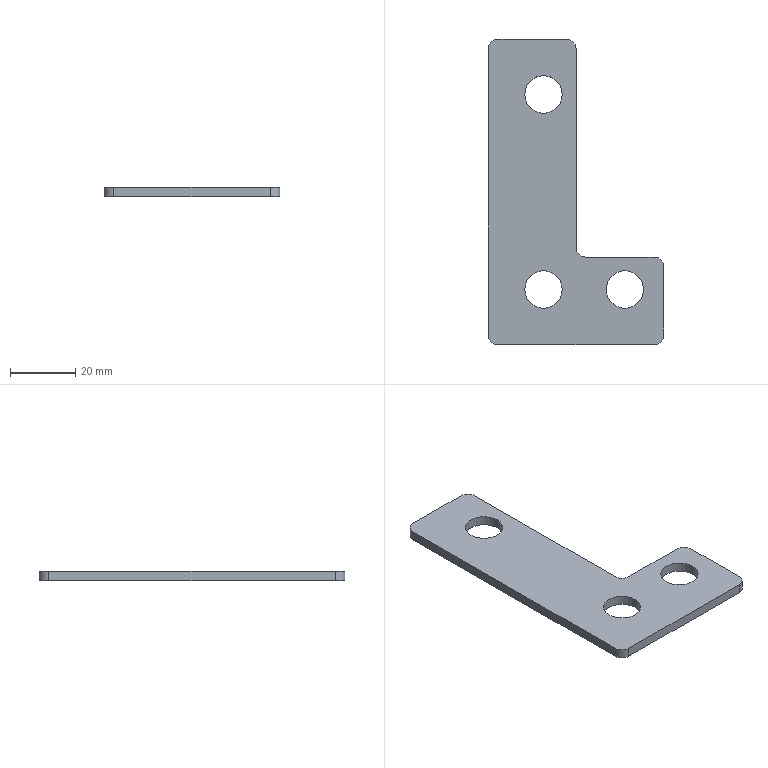Component | SolidWorks | BottomBeamAssembly-1_BottomFrameCornerConnection-1 | 1 solid | 20 faces | box 54 x 94 x 3 mm | volume 8843 mm3 | cylinder 12 | plane 8 | commonest cylinder face diameters 11.5 x6 6 x6
STEP:
#1=COLOUR_RGB('',0.7922,0.8196,0.9333);
#2=FILL_AREA_STYLE_COLOUR('',#1);
#3=FILL_AREA_STYLE('',(#2));
#4=SURFACE_STYLE_FILL_AREA(#3);
#5=SURFACE_SIDE_STYLE('',(#4));
#6=SURFACE_STYLE_USAGE(.BOTH.,#5);
#7=PRESENTATION_STYLE_ASSIGNMENT((#6));
#8=CARTESIAN_POINT('',(-15.865,3.035,-21.339));
#9=VERTEX_POINT('',#8);
#10=CARTESIAN_POINT('',(-15.412,3.035,-21.339));
#11=VERTEX_POINT('',#10);
#12=CARTESIAN_POINT('',(-15.638,3.035,-21.339));
#13=DIRECTION('',(0.,0.,1.));
#14=DIRECTION('',(1.,0.,0.));
#15=AXIS2_PLACEMENT_3D('',#12,#13,#14);
#16=CIRCLE('',#15,0.2264);
#17=EDGE_CURVE('',#9,#11,#16,.T.);
#18=ORIENTED_EDGE('',*,*,#17,.F.);
#19=CARTESIAN_POINT('',(-15.865,3.035,-21.22));
#20=VERTEX_POINT('',#19);
#21=CARTESIAN_POINT('',(-15.865,3.035,-21.614));
#22=DIRECTION('',(0.,0.,1.));
#23=VECTOR('',#22,39.37);
#24=LINE('',#21,#23);
#25=EDGE_CURVE('',#9,#20,#24,.T.);
#26=ORIENTED_EDGE('',*,*,#25,.T.);
#27=CARTESIAN_POINT('',(-15.412,3.035,-21.22));
#28=VERTEX_POINT('',#27);
#29=CARTESIAN_POINT('',(-15.638,3.035,-21.22));
#30=DIRECTION('',(0.,0.,1.));
#31=DIRECTION('',(1.,0.,0.));
#32=AXIS2_PLACEMENT_3D('',#29,#30,#31);
#33=CIRCLE('',#32,0.2264);
#34=EDGE_CURVE('',#20,#28,#33,.T.);
#35=ORIENTED_EDGE('',*,*,#34,.T.);
#36=CARTESIAN_POINT('',(-15.412,3.035,-21.614));
#37=DIRECTION('',(0.,0.,1.));
#38=VECTOR('',#37,39.37);
#39=LINE('',#36,#38);
#40=EDGE_CURVE('',#11,#28,#39,.T.);
#41=ORIENTED_EDGE('',*,*,#40,.F.);
#42=EDGE_LOOP('',(#18,#26,#35,#41));
#43=FACE_OUTER_BOUND('',#42,.T.);
#44=CARTESIAN_POINT('',(-15.638,3.035,-21.614));
#45=DIRECTION('',(0.,0.,1.));
#46=DIRECTION('',(1.,0.,0.));
#47=AXIS2_PLACEMENT_3D('',#44,#45,#46);
#48=CYLINDRICAL_SURFACE('',#47,0.2264);
#49=ADVANCED_FACE('',(#43),#48,.F.);
#50=CARTESIAN_POINT('',(-14.881,0.6732,-21.339));
#51=VERTEX_POINT('',#50);
#52=CARTESIAN_POINT('',(-14.428,0.6732,-21.339));
#53=VERTEX_POINT('',#52);
#54=CARTESIAN_POINT('',(-14.654,0.6732,-21.339));
#55=DIRECTION('',(0.,0.,1.));
#56=DIRECTION('',(1.,0.,0.));
#57=AXIS2_PLACEMENT_3D('',#54,#55,#56);
#58=CIRCLE('',#57,0.2264);
#59=EDGE_CURVE('',#51,#53,#58,.T.);
#60=ORIENTED_EDGE('',*,*,#59,.F.);
#61=CARTESIAN_POINT('',(-14.881,0.6732,-21.22));
#62=VERTEX_POINT('',#61);
#63=CARTESIAN_POINT('',(-14.881,0.6732,-21.614));
#64=DIRECTION('',(0.,0.,1.));
#65=VECTOR('',#64,39.37);
#66=LINE('',#63,#65);
#67=EDGE_CURVE('',#51,#62,#66,.T.);
#68=ORIENTED_EDGE('',*,*,#67,.T.);
#69=CARTESIAN_POINT('',(-14.428,0.6732,-21.22));
#70=VERTEX_POINT('',#69);
#71=CARTESIAN_POINT('',(-14.654,0.6732,-21.22));
#72=DIRECTION('',(0.,0.,1.));
#73=DIRECTION('',(1.,0.,0.));
#74=AXIS2_PLACEMENT_3D('',#71,#72,#73);
#75=CIRCLE('',#74,0.2264);
#76=EDGE_CURVE('',#62,#70,#75,.T.);
#77=ORIENTED_EDGE('',*,*,#76,.T.);
#78=CARTESIAN_POINT('',(-14.428,0.6732,-21.614));
#79=DIRECTION('',(0.,0.,1.));
#80=VECTOR('',#79,39.37);
#81=LINE('',#78,#80);
#82=EDGE_CURVE('',#53,#70,#81,.T.);
#83=ORIENTED_EDGE('',*,*,#82,.F.);
#84=EDGE_LOOP('',(#60,#68,#77,#83));
#85=FACE_OUTER_BOUND('',#84,.T.);
#86=CARTESIAN_POINT('',(-14.654,0.6732,-21.614));
#87=DIRECTION('',(0.,0.,1.));
#88=DIRECTION('',(1.,0.,0.));
#89=AXIS2_PLACEMENT_3D('',#86,#87,#88);
#90=CYLINDRICAL_SURFACE('',#89,0.2264);
#91=ADVANCED_FACE('',(#85),#90,.F.);
#92=CARTESIAN_POINT('',(-15.865,0.6732,-21.339));
#93=VERTEX_POINT('',#92);
#94=CARTESIAN_POINT('',(-15.412,0.6732,-21.339));
#95=VERTEX_POINT('',#94);
#96=CARTESIAN_POINT('',(-15.638,0.6732,-21.339));
#97=DIRECTION('',(0.,0.,1.));
#98=DIRECTION('',(1.,0.,0.));
#99=AXIS2_PLACEMENT_3D('',#96,#97,#98);
#100=CIRCLE('',#99,0.2264);
#101=EDGE_CURVE('',#93,#95,#100,.T.);
#102=ORIENTED_EDGE('',*,*,#101,.F.);
#103=CARTESIAN_POINT('',(-15.865,0.6732,-21.22));
#104=VERTEX_POINT('',#103);
#105=CARTESIAN_POINT('',(-15.865,0.6732,-21.614));
#106=DIRECTION('',(0.,0.,1.));
#107=VECTOR('',#106,39.37);
#108=LINE('',#105,#107);
#109=EDGE_CURVE('',#93,#104,#108,.T.);
#110=ORIENTED_EDGE('',*,*,#109,.T.);
#111=CARTESIAN_POINT('',(-15.412,0.6732,-21.22));
#112=VERTEX_POINT('',#111);
#113=CARTESIAN_POINT('',(-15.638,0.6732,-21.22));
#114=DIRECTION('',(0.,0.,1.));
#115=DIRECTION('',(1.,0.,0.));
#116=AXIS2_PLACEMENT_3D('',#113,#114,#115);
#117=CIRCLE('',#116,0.2264);
#118=EDGE_CURVE('',#104,#112,#117,.T.);
#119=ORIENTED_EDGE('',*,*,#118,.T.);
#120=CARTESIAN_POINT('',(-15.412,0.6732,-21.614));
#121=DIRECTION('',(0.,0.,1.));
#122=VECTOR('',#121,39.37);
#123=LINE('',#120,#122);
#124=EDGE_CURVE('',#95,#112,#123,.T.);
#125=ORIENTED_EDGE('',*,*,#124,.F.);
#126=EDGE_LOOP('',(#102,#110,#119,#125));
#127=FACE_OUTER_BOUND('',#126,.T.);
#128=CARTESIAN_POINT('',(-15.638,0.6732,-21.614));
#129=DIRECTION('',(0.,0.,1.));
#130=DIRECTION('',(1.,0.,0.));
#131=AXIS2_PLACEMENT_3D('',#128,#129,#130);
#132=CYLINDRICAL_SURFACE('',#131,0.2264);
#133=ADVANCED_FACE('',(#127),#132,.F.);
#134=CARTESIAN_POINT('',(-16.308,3.587,-21.339));
#135=VERTEX_POINT('',#134);
#136=CARTESIAN_POINT('',(-16.308,0.122,-21.339));
#137=VERTEX_POINT('',#136);
#138=CARTESIAN_POINT('',(-16.308,3.705,-21.339));
#139=DIRECTION('',(0.,-1.,0.));
#140=VECTOR('',#139,39.37);
#141=LINE('',#138,#140);
#142=EDGE_CURVE('',#135,#137,#141,.T.);
#143=ORIENTED_EDGE('',*,*,#142,.T.);
#144=CARTESIAN_POINT('',(-16.308,0.122,-21.22));
#145=VERTEX_POINT('',#144);
#146=CARTESIAN_POINT('',(-16.308,0.122,-21.339));
#147=DIRECTION('',(0.,0.,1.));
#148=VECTOR('',#147,39.37);
#149=LINE('',#146,#148);
#150=EDGE_CURVE('',#137,#145,#149,.T.);
#151=ORIENTED_EDGE('',*,*,#150,.T.);
#152=CARTESIAN_POINT('',(-16.308,3.587,-21.22));
#153=VERTEX_POINT('',#152);
#154=CARTESIAN_POINT('',(-16.308,3.705,-21.22));
#155=DIRECTION('',(0.,-1.,0.));
#156=VECTOR('',#155,39.37);
#157=LINE('',#154,#156);
#158=EDGE_CURVE('',#153,#145,#157,.T.);
#159=ORIENTED_EDGE('',*,*,#158,.F.);
#160=CARTESIAN_POINT('',(-16.308,3.587,-21.339));
#161=DIRECTION('',(0.,0.,-1.));
#162=VECTOR('',#161,39.37);
#163=LINE('',#160,#162);
#164=EDGE_CURVE('',#153,#135,#163,.T.);
#165=ORIENTED_EDGE('',*,*,#164,.T.);
#166=EDGE_LOOP('',(#143,#151,#159,#165));
#167=FACE_OUTER_BOUND('',#166,.T.);
#168=CARTESIAN_POINT('',(-16.308,3.705,-21.339));
#169=DIRECTION('',(-1.,-0.,0.));
#170=DIRECTION('',(0.,-1.,0.));
#171=AXIS2_PLACEMENT_3D('',#168,#169,#170);
#172=PLANE('',#171);
#173=ADVANCED_FACE('',(#167),#172,.T.);
#174=CARTESIAN_POINT('',(-15.363,3.705,-21.22));
#175=VERTEX_POINT('',#174);
#176=CARTESIAN_POINT('',(-16.19,3.705,-21.22));
#177=VERTEX_POINT('',#176);
#178=CARTESIAN_POINT('',(-15.245,3.705,-21.22));
#179=DIRECTION('',(-1.,0.,0.));
#180=VECTOR('',#179,39.37);
#181=LINE('',#178,#180);
#182=EDGE_CURVE('',#175,#177,#181,.T.);
#183=ORIENTED_EDGE('',*,*,#182,.F.);
#184=CARTESIAN_POINT('',(-15.363,3.705,-21.339));
#185=VERTEX_POINT('',#184);
#186=CARTESIAN_POINT('',(-15.363,3.705,-21.339));
#187=DIRECTION('',(0.,0.,-1.));
#188=VECTOR('',#187,39.37);
#189=LINE('',#186,#188);
#190=EDGE_CURVE('',#175,#185,#189,.T.);
#191=ORIENTED_EDGE('',*,*,#190,.T.);
#192=CARTESIAN_POINT('',(-16.19,3.705,-21.339));
#193=VERTEX_POINT('',#192);
#194=CARTESIAN_POINT('',(-15.245,3.705,-21.339));
#195=DIRECTION('',(-1.,0.,0.));
#196=VECTOR('',#195,39.37);
#197=LINE('',#194,#196);
#198=EDGE_CURVE('',#185,#193,#197,.T.);
#199=ORIENTED_EDGE('',*,*,#198,.T.);
#200=CARTESIAN_POINT('',(-16.19,3.705,-21.339));
#201=DIRECTION('',(0.,0.,1.));
#202=VECTOR('',#201,39.37);
#203=LINE('',#200,#202);
#204=EDGE_CURVE('',#193,#177,#203,.T.);
#205=ORIENTED_EDGE('',*,*,#204,.T.);
#206=EDGE_LOOP('',(#183,#191,#199,#205));
#207=FACE_OUTER_BOUND('',#206,.T.);
#208=CARTESIAN_POINT('',(-15.245,3.705,-21.339));
#209=DIRECTION('',(0.,1.,0.));
#210=DIRECTION('',(0.,0.,1.));
#211=AXIS2_PLACEMENT_3D('',#208,#209,#210);
#212=PLANE('',#211);
#213=ADVANCED_FACE('',(#207),#212,.T.);
#214=CARTESIAN_POINT('',(-15.245,1.185,-21.22));
#215=VERTEX_POINT('',#214);
#216=CARTESIAN_POINT('',(-15.245,3.587,-21.22));
#217=VERTEX_POINT('',#216);
#218=CARTESIAN_POINT('',(-15.245,1.067,-21.22));
#219=DIRECTION('',(0.,1.,0.));
#220=VECTOR('',#219,39.37);
#221=LINE('',#218,#220);
#222=EDGE_CURVE('',#215,#217,#221,.T.);
#223=ORIENTED_EDGE('',*,*,#222,.F.);
#224=CARTESIAN_POINT('',(-15.245,1.185,-21.339));
#225=VERTEX_POINT('',#224);
#226=CARTESIAN_POINT('',(-15.245,1.185,-21.339));
#227=DIRECTION('',(0.,0.,-1.));
#228=VECTOR('',#227,39.37);
#229=LINE('',#226,#228);
#230=EDGE_CURVE('',#215,#225,#229,.T.);
#231=ORIENTED_EDGE('',*,*,#230,.T.);
#232=CARTESIAN_POINT('',(-15.245,3.587,-21.339));
#233=VERTEX_POINT('',#232);
#234=CARTESIAN_POINT('',(-15.245,1.067,-21.339));
#235=DIRECTION('',(0.,1.,0.));
#236=VECTOR('',#235,39.37);
#237=LINE('',#234,#236);
#238=EDGE_CURVE('',#225,#233,#237,.T.);
#239=ORIENTED_EDGE('',*,*,#238,.T.);
#240=CARTESIAN_POINT('',(-15.245,3.587,-21.339));
#241=DIRECTION('',(0.,0.,1.));
#242=VECTOR('',#241,39.37);
#243=LINE('',#240,#242);
#244=EDGE_CURVE('',#233,#217,#243,.T.);
#245=ORIENTED_EDGE('',*,*,#244,.T.);
#246=EDGE_LOOP('',(#223,#231,#239,#245));
#247=FACE_OUTER_BOUND('',#246,.T.);
#248=CARTESIAN_POINT('',(-15.245,1.067,-21.339));
#249=DIRECTION('',(1.,0.,0.));
#250=DIRECTION('',(0.,0.,-1.));
#251=AXIS2_PLACEMENT_3D('',#248,#249,#250);
#252=PLANE('',#251);
#253=ADVANCED_FACE('',(#247),#252,.T.);
#254=CARTESIAN_POINT('',(-14.3,1.067,-21.339));
#255=VERTEX_POINT('',#254);
#256=CARTESIAN_POINT('',(-15.127,1.067,-21.339));
#257=VERTEX_POINT('',#256);
#258=CARTESIAN_POINT('',(-14.182,1.067,-21.339));
#259=DIRECTION('',(-1.,-0.,0.));
#260=VECTOR('',#259,39.37);
#261=LINE('',#258,#260);
#262=EDGE_CURVE('',#255,#257,#261,.T.);
#263=ORIENTED_EDGE('',*,*,#262,.T.);
#264=CARTESIAN_POINT('',(-15.127,1.067,-21.22));
#265=VERTEX_POINT('',#264);
#266=CARTESIAN_POINT('',(-15.127,1.067,-21.22));
#267=DIRECTION('',(0.,0.,1.));
#268=VECTOR('',#267,39.37);
#269=LINE('',#266,#268);
#270=EDGE_CURVE('',#257,#265,#269,.T.);
#271=ORIENTED_EDGE('',*,*,#270,.T.);
#272=CARTESIAN_POINT('',(-14.3,1.067,-21.22));
#273=VERTEX_POINT('',#272);
#274=CARTESIAN_POINT('',(-14.182,1.067,-21.22));
#275=DIRECTION('',(-1.,-0.,0.));
#276=VECTOR('',#275,39.37);
#277=LINE('',#274,#276);
#278=EDGE_CURVE('',#273,#265,#277,.T.);
#279=ORIENTED_EDGE('',*,*,#278,.F.);
#280=CARTESIAN_POINT('',(-14.3,1.067,-21.339));
#281=DIRECTION('',(0.,0.,-1.));
#282=VECTOR('',#281,39.37);
#283=LINE('',#280,#282);
#284=EDGE_CURVE('',#273,#255,#283,.T.);
#285=ORIENTED_EDGE('',*,*,#284,.T.);
#286=EDGE_LOOP('',(#263,#271,#279,#285));
#287=FACE_OUTER_BOUND('',#286,.T.);
#288=CARTESIAN_POINT('',(-14.182,1.067,-21.339));
#289=DIRECTION('',(-0.,1.,0.));
#290=DIRECTION('',(-1.,-0.,0.));
#291=AXIS2_PLACEMENT_3D('',#288,#289,#290);
#292=PLANE('',#291);
#293=ADVANCED_FACE('',(#287),#292,.T.);
#294=CARTESIAN_POINT('',(-14.182,0.122,-21.22));
#295=VERTEX_POINT('',#294);
#296=CARTESIAN_POINT('',(-14.182,0.9488,-21.22));
#297=VERTEX_POINT('',#296);
#298=CARTESIAN_POINT('',(-14.182,0.003927,-21.22));
#299=DIRECTION('',(0.,1.,0.));
#300=VECTOR('',#299,39.37);
#301=LINE('',#298,#300);
#302=EDGE_CURVE('',#295,#297,#301,.T.);
#303=ORIENTED_EDGE('',*,*,#302,.F.);
#304=CARTESIAN_POINT('',(-14.182,0.122,-21.339));
#305=VERTEX_POINT('',#304);
#306=CARTESIAN_POINT('',(-14.182,0.122,-21.339));
#307=DIRECTION('',(0.,0.,-1.));
#308=VECTOR('',#307,39.37);
#309=LINE('',#306,#308);
#310=EDGE_CURVE('',#295,#305,#309,.T.);
#311=ORIENTED_EDGE('',*,*,#310,.T.);
#312=CARTESIAN_POINT('',(-14.182,0.9488,-21.339));
#313=VERTEX_POINT('',#312);
#314=CARTESIAN_POINT('',(-14.182,0.003927,-21.339));
#315=DIRECTION('',(0.,1.,0.));
#316=VECTOR('',#315,39.37);
#317=LINE('',#314,#316);
#318=EDGE_CURVE('',#305,#313,#317,.T.);
#319=ORIENTED_EDGE('',*,*,#318,.T.);
#320=CARTESIAN_POINT('',(-14.182,0.9488,-21.339));
#321=DIRECTION('',(0.,0.,1.));
#322=VECTOR('',#321,39.37);
#323=LINE('',#320,#322);
#324=EDGE_CURVE('',#313,#297,#323,.T.);
#325=ORIENTED_EDGE('',*,*,#324,.T.);
#326=EDGE_LOOP('',(#303,#311,#319,#325));
#327=FACE_OUTER_BOUND('',#326,.T.);
#328=CARTESIAN_POINT('',(-14.182,0.003927,-21.339));
#329=DIRECTION('',(1.,0.,0.));
#330=DIRECTION('',(0.,0.,-1.));
#331=AXIS2_PLACEMENT_3D('',#328,#329,#330);
#332=PLANE('',#331);
#333=ADVANCED_FACE('',(#327),#332,.T.);
#334=CARTESIAN_POINT('',(-16.19,0.003927,-21.22));
#335=VERTEX_POINT('',#334);
#336=CARTESIAN_POINT('',(-14.3,0.003927,-21.22));
#337=VERTEX_POINT('',#336);
#338=CARTESIAN_POINT('',(-16.308,0.003927,-21.22));
#339=DIRECTION('',(1.,0.,0.));
#340=VECTOR('',#339,39.37);
#341=LINE('',#338,#340);
#342=EDGE_CURVE('',#335,#337,#341,.T.);
#343=ORIENTED_EDGE('',*,*,#342,.F.);
#344=CARTESIAN_POINT('',(-16.19,0.003927,-21.339));
#345=VERTEX_POINT('',#344);
#346=CARTESIAN_POINT('',(-16.19,0.003927,-21.339));
#347=DIRECTION('',(0.,0.,-1.));
#348=VECTOR('',#347,39.37);
#349=LINE('',#346,#348);
#350=EDGE_CURVE('',#335,#345,#349,.T.);
#351=ORIENTED_EDGE('',*,*,#350,.T.);
#352=CARTESIAN_POINT('',(-14.3,0.003927,-21.339));
#353=VERTEX_POINT('',#352);
#354=CARTESIAN_POINT('',(-16.308,0.003927,-21.339));
#355=DIRECTION('',(1.,0.,0.));
#356=VECTOR('',#355,39.37);
#357=LINE('',#354,#356);
#358=EDGE_CURVE('',#345,#353,#357,.T.);
#359=ORIENTED_EDGE('',*,*,#358,.T.);
#360=CARTESIAN_POINT('',(-14.3,0.003927,-21.339));
#361=DIRECTION('',(0.,0.,1.));
#362=VECTOR('',#361,39.37);
#363=LINE('',#360,#362);
#364=EDGE_CURVE('',#353,#337,#363,.T.);
#365=ORIENTED_EDGE('',*,*,#364,.T.);
#366=EDGE_LOOP('',(#343,#351,#359,#365));
#367=FACE_OUTER_BOUND('',#366,.T.);
#368=CARTESIAN_POINT('',(-16.308,0.003927,-21.339));
#369=DIRECTION('',(0.,-1.,0.));
#370=DIRECTION('',(0.,0.,-1.));
#371=AXIS2_PLACEMENT_3D('',#368,#369,#370);
#372=PLANE('',#371);
#373=ADVANCED_FACE('',(#367),#372,.T.);
#374=CARTESIAN_POINT('',(-15.638,3.035,-21.339));
#375=DIRECTION('',(0.,0.,1.));
#376=DIRECTION('',(1.,0.,0.));
#377=AXIS2_PLACEMENT_3D('',#374,#375,#376);
#378=CIRCLE('',#377,0.2264);
#379=EDGE_CURVE('',#11,#9,#378,.T.);
#380=ORIENTED_EDGE('',*,*,#379,.T.);
#381=ORIENTED_EDGE('',*,*,#17,.T.);
#382=EDGE_LOOP('',(#380,#381));
#383=FACE_BOUND('',#382,.T.);
#384=CARTESIAN_POINT('',(-14.654,0.6732,-21.339));
#385=DIRECTION('',(0.,0.,1.));
#386=DIRECTION('',(1.,0.,0.));
#387=AXIS2_PLACEMENT_3D('',#384,#385,#386);
#388=CIRCLE('',#387,0.2264);
#389=EDGE_CURVE('',#53,#51,#388,.T.);
#390=ORIENTED_EDGE('',*,*,#389,.T.);
#391=ORIENTED_EDGE('',*,*,#59,.T.);
#392=EDGE_LOOP('',(#390,#391));
#393=FACE_BOUND('',#392,.T.);
#394=CARTESIAN_POINT('',(-15.638,0.6732,-21.339));
#395=DIRECTION('',(0.,0.,1.));
#396=DIRECTION('',(1.,0.,0.));
#397=AXIS2_PLACEMENT_3D('',#394,#395,#396);
#398=CIRCLE('',#397,0.2264);
#399=EDGE_CURVE('',#95,#93,#398,.T.);
#400=ORIENTED_EDGE('',*,*,#399,.T.);
#401=ORIENTED_EDGE('',*,*,#101,.T.);
#402=EDGE_LOOP('',(#400,#401));
#403=FACE_BOUND('',#402,.T.);
#404=ORIENTED_EDGE('',*,*,#358,.F.);
#405=CARTESIAN_POINT('',(-16.19,0.122,-21.339));
#406=DIRECTION('',(0.,0.,-1.));
#407=DIRECTION('',(1.,0.,0.));
#408=AXIS2_PLACEMENT_3D('',#405,#406,#407);
#409=CIRCLE('',#408,0.1181);
#410=EDGE_CURVE('',#345,#137,#409,.T.);
#411=ORIENTED_EDGE('',*,*,#410,.T.);
#412=ORIENTED_EDGE('',*,*,#142,.F.);
#413=CARTESIAN_POINT('',(-16.19,3.587,-21.339));
#414=DIRECTION('',(0.,0.,-1.));
#415=DIRECTION('',(1.,0.,0.));
#416=AXIS2_PLACEMENT_3D('',#413,#414,#415);
#417=CIRCLE('',#416,0.1181);
#418=EDGE_CURVE('',#135,#193,#417,.T.);
#419=ORIENTED_EDGE('',*,*,#418,.T.);
#420=ORIENTED_EDGE('',*,*,#198,.F.);
#421=CARTESIAN_POINT('',(-15.363,3.587,-21.339));
#422=DIRECTION('',(0.,0.,-1.));
#423=DIRECTION('',(1.,0.,0.));
#424=AXIS2_PLACEMENT_3D('',#421,#422,#423);
#425=CIRCLE('',#424,0.1181);
#426=EDGE_CURVE('',#185,#233,#425,.T.);
#427=ORIENTED_EDGE('',*,*,#426,.T.);
#428=ORIENTED_EDGE('',*,*,#238,.F.);
#429=CARTESIAN_POINT('',(-15.127,1.185,-21.339));
#430=DIRECTION('',(0.,0.,1.));
#431=DIRECTION('',(1.,0.,0.));
#432=AXIS2_PLACEMENT_3D('',#429,#430,#431);
#433=CIRCLE('',#432,0.1181);
#434=EDGE_CURVE('',#225,#257,#433,.T.);
#435=ORIENTED_EDGE('',*,*,#434,.T.);
#436=ORIENTED_EDGE('',*,*,#262,.F.);
#437=CARTESIAN_POINT('',(-14.3,0.9488,-21.339));
#438=DIRECTION('',(0.,0.,-1.));
#439=DIRECTION('',(1.,0.,0.));
#440=AXIS2_PLACEMENT_3D('',#437,#438,#439);
#441=CIRCLE('',#440,0.1181);
#442=EDGE_CURVE('',#255,#313,#441,.T.);
#443=ORIENTED_EDGE('',*,*,#442,.T.);
#444=ORIENTED_EDGE('',*,*,#318,.F.);
#445=CARTESIAN_POINT('',(-14.3,0.122,-21.339));
#446=DIRECTION('',(0.,0.,-1.));
#447=DIRECTION('',(1.,0.,0.));
#448=AXIS2_PLACEMENT_3D('',#445,#446,#447);
#449=CIRCLE('',#448,0.1181);
#450=EDGE_CURVE('',#305,#353,#449,.T.);
#451=ORIENTED_EDGE('',*,*,#450,.T.);
#452=EDGE_LOOP('',(#404,#411,#412,#419,#420,#427,#428,#435,#436,#443,#444,#451));
#453=FACE_OUTER_BOUND('',#452,.T.);
#454=CARTESIAN_POINT('',(-16.308,0.003927,-21.339));
#455=DIRECTION('',(0.,0.,1.));
#456=DIRECTION('',(1.,0.,0.));
#457=AXIS2_PLACEMENT_3D('',#454,#455,#456);
#458=PLANE('',#457);
#459=ADVANCED_FACE('',(#383,#393,#403,#453),#458,.F.);
#460=CARTESIAN_POINT('',(-15.638,3.035,-21.22));
#461=DIRECTION('',(0.,0.,1.));
#462=DIRECTION('',(1.,0.,0.));
#463=AXIS2_PLACEMENT_3D('',#460,#461,#462);
#464=CIRCLE('',#463,0.2264);
#465=EDGE_CURVE('',#28,#20,#464,.T.);
#466=ORIENTED_EDGE('',*,*,#465,.F.);
#467=ORIENTED_EDGE('',*,*,#34,.F.);
#468=EDGE_LOOP('',(#466,#467));
#469=FACE_BOUND('',#468,.T.);
#470=CARTESIAN_POINT('',(-14.654,0.6732,-21.22));
#471=DIRECTION('',(0.,0.,1.));
#472=DIRECTION('',(1.,0.,0.));
#473=AXIS2_PLACEMENT_3D('',#470,#471,#472);
#474=CIRCLE('',#473,0.2264);
#475=EDGE_CURVE('',#70,#62,#474,.T.);
#476=ORIENTED_EDGE('',*,*,#475,.F.);
#477=ORIENTED_EDGE('',*,*,#76,.F.);
#478=EDGE_LOOP('',(#476,#477));
#479=FACE_BOUND('',#478,.T.);
#480=CARTESIAN_POINT('',(-15.638,0.6732,-21.22));
#481=DIRECTION('',(0.,0.,1.));
#482=DIRECTION('',(1.,0.,0.));
#483=AXIS2_PLACEMENT_3D('',#480,#481,#482);
#484=CIRCLE('',#483,0.2264);
#485=EDGE_CURVE('',#112,#104,#484,.T.);
#486=ORIENTED_EDGE('',*,*,#485,.F.);
#487=ORIENTED_EDGE('',*,*,#118,.F.);
#488=EDGE_LOOP('',(#486,#487));
#489=FACE_BOUND('',#488,.T.);
#490=ORIENTED_EDGE('',*,*,#158,.T.);
#491=CARTESIAN_POINT('',(-16.19,0.122,-21.22));
#492=DIRECTION('',(0.,0.,1.));
#493=DIRECTION('',(1.,0.,0.));
#494=AXIS2_PLACEMENT_3D('',#491,#492,#493);
#495=CIRCLE('',#494,0.1181);
#496=EDGE_CURVE('',#145,#335,#495,.T.);
#497=ORIENTED_EDGE('',*,*,#496,.T.);
#498=ORIENTED_EDGE('',*,*,#342,.T.);
#499=CARTESIAN_POINT('',(-14.3,0.122,-21.22));
#500=DIRECTION('',(0.,0.,1.));
#501=DIRECTION('',(1.,0.,0.));
#502=AXIS2_PLACEMENT_3D('',#499,#500,#501);
#503=CIRCLE('',#502,0.1181);
#504=EDGE_CURVE('',#337,#295,#503,.T.);
#505=ORIENTED_EDGE('',*,*,#504,.T.);
#506=ORIENTED_EDGE('',*,*,#302,.T.);
#507=CARTESIAN_POINT('',(-14.3,0.9488,-21.22));
#508=DIRECTION('',(0.,0.,1.));
#509=DIRECTION('',(1.,0.,0.));
#510=AXIS2_PLACEMENT_3D('',#507,#508,#509);
#511=CIRCLE('',#510,0.1181);
#512=EDGE_CURVE('',#297,#273,#511,.T.);
#513=ORIENTED_EDGE('',*,*,#512,.T.);
#514=ORIENTED_EDGE('',*,*,#278,.T.);
#515=CARTESIAN_POINT('',(-15.127,1.185,-21.22));
#516=DIRECTION('',(0.,0.,-1.));
#517=DIRECTION('',(1.,0.,0.));
#518=AXIS2_PLACEMENT_3D('',#515,#516,#517);
#519=CIRCLE('',#518,0.1181);
#520=EDGE_CURVE('',#265,#215,#519,.T.);
#521=ORIENTED_EDGE('',*,*,#520,.T.);
#522=ORIENTED_EDGE('',*,*,#222,.T.);
#523=CARTESIAN_POINT('',(-15.363,3.587,-21.22));
#524=DIRECTION('',(0.,0.,1.));
#525=DIRECTION('',(1.,0.,0.));
#526=AXIS2_PLACEMENT_3D('',#523,#524,#525);
#527=CIRCLE('',#526,0.1181);
#528=EDGE_CURVE('',#217,#175,#527,.T.);
#529=ORIENTED_EDGE('',*,*,#528,.T.);
#530=ORIENTED_EDGE('',*,*,#182,.T.);
#531=CARTESIAN_POINT('',(-16.19,3.587,-21.22));
#532=DIRECTION('',(0.,0.,1.));
#533=DIRECTION('',(1.,0.,0.));
#534=AXIS2_PLACEMENT_3D('',#531,#532,#533);
#535=CIRCLE('',#534,0.1181);
#536=EDGE_CURVE('',#177,#153,#535,.T.);
#537=ORIENTED_EDGE('',*,*,#536,.T.);
#538=EDGE_LOOP('',(#490,#497,#498,#505,#506,#513,#514,#521,#522,#529,#530,#537));
#539=FACE_OUTER_BOUND('',#538,.T.);
#540=CARTESIAN_POINT('',(-16.308,0.003927,-21.22));
#541=DIRECTION('',(0.,0.,1.));
#542=DIRECTION('',(1.,0.,0.));
#543=AXIS2_PLACEMENT_3D('',#540,#541,#542);
#544=PLANE('',#543);
#545=ADVANCED_FACE('',(#469,#479,#489,#539),#544,.T.);
#546=ORIENTED_EDGE('',*,*,#434,.F.);
#547=ORIENTED_EDGE('',*,*,#230,.F.);
#548=ORIENTED_EDGE('',*,*,#520,.F.);
#549=ORIENTED_EDGE('',*,*,#270,.F.);
#550=EDGE_LOOP('',(#546,#547,#548,#549));
#551=FACE_OUTER_BOUND('',#550,.T.);
#552=CARTESIAN_POINT('',(-15.127,1.185,-21.339));
#553=DIRECTION('',(0.,0.,-1.));
#554=DIRECTION('',(-1.,0.,0.));
#555=AXIS2_PLACEMENT_3D('',#552,#553,#554);
#556=CYLINDRICAL_SURFACE('',#555,0.1181);
#557=ADVANCED_FACE('',(#551),#556,.F.);
#558=ORIENTED_EDGE('',*,*,#410,.F.);
#559=ORIENTED_EDGE('',*,*,#350,.F.);
#560=ORIENTED_EDGE('',*,*,#496,.F.);
#561=ORIENTED_EDGE('',*,*,#150,.F.);
#562=EDGE_LOOP('',(#558,#559,#560,#561));
#563=FACE_OUTER_BOUND('',#562,.T.);
#564=CARTESIAN_POINT('',(-16.19,0.122,-21.339));
#565=DIRECTION('',(0.,0.,1.));
#566=DIRECTION('',(1.,0.,0.));
#567=AXIS2_PLACEMENT_3D('',#564,#565,#566);
#568=CYLINDRICAL_SURFACE('',#567,0.1181);
#569=ADVANCED_FACE('',(#563),#568,.T.);
#570=ORIENTED_EDGE('',*,*,#450,.F.);
#571=ORIENTED_EDGE('',*,*,#310,.F.);
#572=ORIENTED_EDGE('',*,*,#504,.F.);
#573=ORIENTED_EDGE('',*,*,#364,.F.);
#574=EDGE_LOOP('',(#570,#571,#572,#573));
#575=FACE_OUTER_BOUND('',#574,.T.);
#576=CARTESIAN_POINT('',(-14.3,0.122,-21.339));
#577=DIRECTION('',(0.,0.,1.));
#578=DIRECTION('',(1.,0.,0.));
#579=AXIS2_PLACEMENT_3D('',#576,#577,#578);
#580=CYLINDRICAL_SURFACE('',#579,0.1181);
#581=ADVANCED_FACE('',(#575),#580,.T.);
#582=ORIENTED_EDGE('',*,*,#442,.F.);
#583=ORIENTED_EDGE('',*,*,#284,.F.);
#584=ORIENTED_EDGE('',*,*,#512,.F.);
#585=ORIENTED_EDGE('',*,*,#324,.F.);
#586=EDGE_LOOP('',(#582,#583,#584,#585));
#587=FACE_OUTER_BOUND('',#586,.T.);
#588=CARTESIAN_POINT('',(-14.3,0.9488,-21.339));
#589=DIRECTION('',(0.,0.,1.));
#590=DIRECTION('',(1.,0.,0.));
#591=AXIS2_PLACEMENT_3D('',#588,#589,#590);
#592=CYLINDRICAL_SURFACE('',#591,0.1181);
#593=ADVANCED_FACE('',(#587),#592,.T.);
#594=ORIENTED_EDGE('',*,*,#426,.F.);
#595=ORIENTED_EDGE('',*,*,#190,.F.);
#596=ORIENTED_EDGE('',*,*,#528,.F.);
#597=ORIENTED_EDGE('',*,*,#244,.F.);
#598=EDGE_LOOP('',(#594,#595,#596,#597));
#599=FACE_OUTER_BOUND('',#598,.T.);
#600=CARTESIAN_POINT('',(-15.363,3.587,-21.339));
#601=DIRECTION('',(0.,0.,1.));
#602=DIRECTION('',(1.,0.,0.));
#603=AXIS2_PLACEMENT_3D('',#600,#601,#602);
#604=CYLINDRICAL_SURFACE('',#603,0.1181);
#605=ADVANCED_FACE('',(#599),#604,.T.);
#606=ORIENTED_EDGE('',*,*,#418,.F.);
#607=ORIENTED_EDGE('',*,*,#164,.F.);
#608=ORIENTED_EDGE('',*,*,#536,.F.);
#609=ORIENTED_EDGE('',*,*,#204,.F.);
#610=EDGE_LOOP('',(#606,#607,#608,#609));
#611=FACE_OUTER_BOUND('',#610,.T.);
#612=CARTESIAN_POINT('',(-16.19,3.587,-21.339));
#613=DIRECTION('',(0.,0.,1.));
#614=DIRECTION('',(1.,0.,0.));
#615=AXIS2_PLACEMENT_3D('',#612,#613,#614);
#616=CYLINDRICAL_SURFACE('',#615,0.1181);
#617=ADVANCED_FACE('',(#611),#616,.T.);
#618=ORIENTED_EDGE('',*,*,#109,.F.);
#619=ORIENTED_EDGE('',*,*,#399,.F.);
#620=ORIENTED_EDGE('',*,*,#124,.T.);
#621=ORIENTED_EDGE('',*,*,#485,.T.);
#622=EDGE_LOOP('',(#618,#619,#620,#621));
#623=FACE_OUTER_BOUND('',#622,.T.);
#624=CARTESIAN_POINT('',(-15.638,0.6732,-21.614));
#625=DIRECTION('',(0.,0.,1.));
#626=DIRECTION('',(1.,0.,0.));
#627=AXIS2_PLACEMENT_3D('',#624,#625,#626);
#628=CYLINDRICAL_SURFACE('',#627,0.2264);
#629=ADVANCED_FACE('',(#623),#628,.F.);
#630=ORIENTED_EDGE('',*,*,#67,.F.);
#631=ORIENTED_EDGE('',*,*,#389,.F.);
#632=ORIENTED_EDGE('',*,*,#82,.T.);
#633=ORIENTED_EDGE('',*,*,#475,.T.);
#634=EDGE_LOOP('',(#630,#631,#632,#633));
#635=FACE_OUTER_BOUND('',#634,.T.);
#636=CARTESIAN_POINT('',(-14.654,0.6732,-21.614));
#637=DIRECTION('',(0.,0.,1.));
#638=DIRECTION('',(1.,0.,0.));
#639=AXIS2_PLACEMENT_3D('',#636,#637,#638);
#640=CYLINDRICAL_SURFACE('',#639,0.2264);
#641=ADVANCED_FACE('',(#635),#640,.F.);
#642=ORIENTED_EDGE('',*,*,#25,.F.);
#643=ORIENTED_EDGE('',*,*,#379,.F.);
#644=ORIENTED_EDGE('',*,*,#40,.T.);
#645=ORIENTED_EDGE('',*,*,#465,.T.);
#646=EDGE_LOOP('',(#642,#643,#644,#645));
#647=FACE_OUTER_BOUND('',#646,.T.);
#648=CARTESIAN_POINT('',(-15.638,3.035,-21.614));
#649=DIRECTION('',(0.,0.,1.));
#650=DIRECTION('',(1.,0.,0.));
#651=AXIS2_PLACEMENT_3D('',#648,#649,#650);
#652=CYLINDRICAL_SURFACE('',#651,0.2264);
#653=ADVANCED_FACE('',(#647),#652,.F.);
#654=CLOSED_SHELL('',(#49,#91,#133,#173,#213,#253,#293,#333,#373,#459,#545,#557,#569,#581,#593,#605,#617,#629,#641,#653));
#655=MANIFOLD_SOLID_BREP('',#654);
#656=STYLED_ITEM('',(#7),#655);
#657=PRESENTATION_LAYER_ASSIGNMENT('','',(#656));
#658=(LENGTH_UNIT()NAMED_UNIT(*)SI_UNIT($,.METRE.));
#659=LENGTH_MEASURE_WITH_UNIT(LENGTH_MEASURE(0.0254),#658);
#660=DIMENSIONAL_EXPONENTS(1.,0.,0.,0.,0.,0.,0.);
#661=(CONVERSION_BASED_UNIT('',#659)LENGTH_UNIT()NAMED_UNIT(#660));
#662=UNCERTAINTY_MEASURE_WITH_UNIT(LENGTH_MEASURE(0.00001),#661,'','');
#663=(NAMED_UNIT(*)PLANE_ANGLE_UNIT()SI_UNIT($,.RADIAN.));
#664=(NAMED_UNIT(*)SI_UNIT($,.STERADIAN.)SOLID_ANGLE_UNIT());
#665=(GEOMETRIC_REPRESENTATION_CONTEXT(3)GLOBAL_UNCERTAINTY_ASSIGNED_CONTEXT((#662))GLOBAL_UNIT_ASSIGNED_CONTEXT((#661,#663,#664))REPRESENTATION_CONTEXT('',''));
#666=MECHANICAL_DESIGN_GEOMETRIC_PRESENTATION_REPRESENTATION('',(#656),#665);
#667=CARTESIAN_POINT('',(0.,0.,0.));
#668=DIRECTION('',(0.,0.,1.));
#669=DIRECTION('',(1.,0.,0.));
#670=AXIS2_PLACEMENT_3D('',#667,#668,#669);
#671=(LENGTH_UNIT()NAMED_UNIT(*)SI_UNIT($,.METRE.));
#672=LENGTH_MEASURE_WITH_UNIT(LENGTH_MEASURE(0.0254),#671);
#673=DIMENSIONAL_EXPONENTS(1.,0.,0.,0.,0.,0.,0.);
#674=(CONVERSION_BASED_UNIT('',#672)LENGTH_UNIT()NAMED_UNIT(#673));
#675=UNCERTAINTY_MEASURE_WITH_UNIT(LENGTH_MEASURE(0.00001),#674,'','');
#676=(NAMED_UNIT(*)PLANE_ANGLE_UNIT()SI_UNIT($,.RADIAN.));
#677=(NAMED_UNIT(*)SI_UNIT($,.STERADIAN.)SOLID_ANGLE_UNIT());
#678=(GEOMETRIC_REPRESENTATION_CONTEXT(3)GLOBAL_UNCERTAINTY_ASSIGNED_CONTEXT((#675))GLOBAL_UNIT_ASSIGNED_CONTEXT((#674,#676,#677))REPRESENTATION_CONTEXT('',''));
#679=ADVANCED_BREP_SHAPE_REPRESENTATION('',(#655,#670),#678);